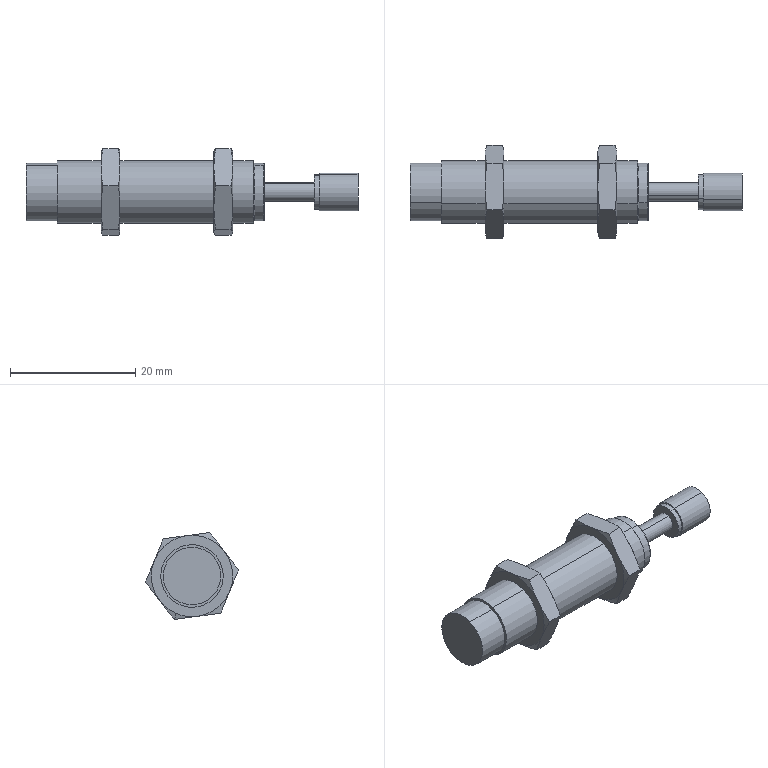Component | SolidWorks | Buffer-1 | 1 solid | 70 faces | box 53 x 14.88 x 13.87 mm | volume 3558 mm3 | cone 32 | plane 22 | cylinder 16 | commonest cylinder face diameters 10 x6 9.2 x4 6 x2 5.6 x2 3 x2